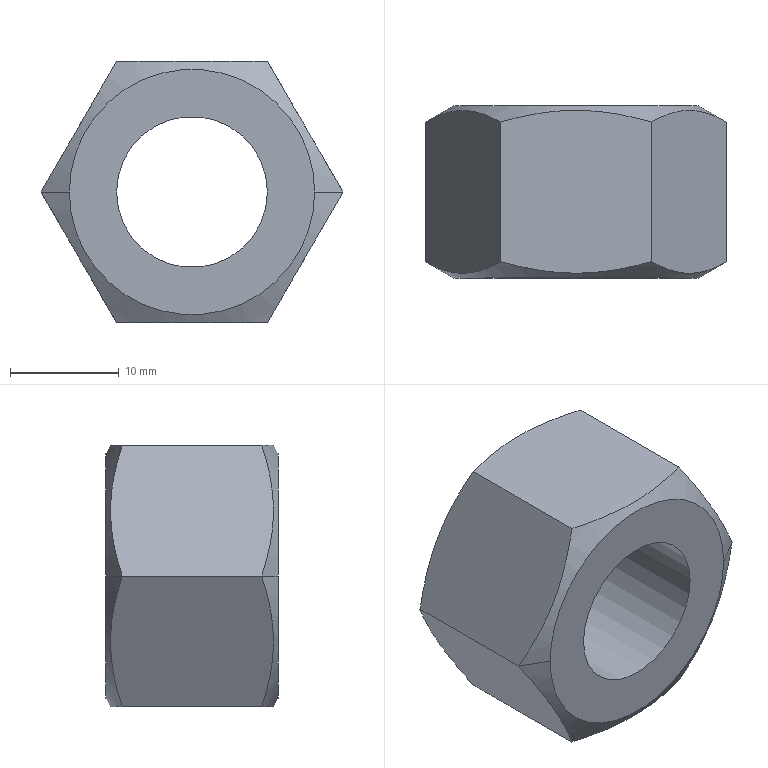Component | SolidWorks | m16-3 | 1 solid | 14 faces | box 27.71 x 15.8 x 24 mm | volume 5411 mm3 | plane 8 | cone 4 | cylinder 2 | commonest cylinder face diameters 13.84 x2
build123d program:
from build123d import *

# Parameters (mm, degrees)
BOSS_EXTRUDE1_DEPTH = 15.8
SKETCH3_R           = 6.92
CUT_EXTRUDE1_DEPTH  = 25.2


with BuildPart() as part:
    # Sketch1 → Boss-Extrude1 (new body)
    with BuildSketch(Plane.XY):
        Polygon((13.856, 0), (6.928, 12), (-6.928, 12), (-13.856, 0), (-6.928, -12), (6.928, -12), align=None)
    extrude(amount=BOSS_EXTRUDE1_DEPTH)

    # Sketch2 → Cut-Revolve1 (revolve, cut)
    with BuildSketch(Plane(origin=(0, 0, 0), x_dir=(1, 0, 0), z_dir=(0, 1, 0))):
        Polygon((13.856, -1.5), (6.928, 2.5), (16.856, 3.696), align=None)
        Polygon((13.856, -14.3), (6.928, -18.3), (16.856, -19.496), align=None)
    revolve(axis=Axis((0, 0, 0), (0, 0, 1)), mode=Mode.SUBTRACT)

    # Sketch3 → Cut-Extrude1 (cut, through all)
    with BuildSketch(Plane.XY):
        Circle(SKETCH3_R)
    extrude(amount=CUT_EXTRUDE1_DEPTH, mode=Mode.SUBTRACT)


solid = part.part

# Placed as in the assembly
solid = solid.moved(Location((726.83, 1299.391, 1682.217), (90, 0, 0)))
STEP:
#1=COLOUR_RGB('',0.7922,0.8196,0.9333);
#2=FILL_AREA_STYLE_COLOUR('',#1);
#3=FILL_AREA_STYLE('',(#2));
#4=SURFACE_STYLE_FILL_AREA(#3);
#5=SURFACE_SIDE_STYLE('',(#4));
#6=SURFACE_STYLE_USAGE(.BOTH.,#5);
#7=PRESENTATION_STYLE_ASSIGNMENT((#6));
#8=CARTESIAN_POINT('',(28.343,50.535,66.229));
#9=VERTEX_POINT('',#8);
#10=CARTESIAN_POINT('',(28.888,50.535,66.229));
#11=VERTEX_POINT('',#10);
#12=CARTESIAN_POINT('',(28.615,50.535,66.229));
#13=DIRECTION('',(0.,-1.,0.));
#14=DIRECTION('',(1.,0.,0.));
#15=AXIS2_PLACEMENT_3D('',#12,#13,#14);
#16=CIRCLE('',#15,0.2724);
#17=EDGE_CURVE('',#9,#11,#16,.T.);
#18=ORIENTED_EDGE('',*,*,#17,.T.);
#19=CARTESIAN_POINT('',(28.888,51.157,66.229));
#20=VERTEX_POINT('',#19);
#21=CARTESIAN_POINT('',(28.888,50.535,66.229));
#22=DIRECTION('',(0.,1.,0.));
#23=VECTOR('',#22,39.37);
#24=LINE('',#21,#23);
#25=EDGE_CURVE('',#11,#20,#24,.T.);
#26=ORIENTED_EDGE('',*,*,#25,.T.);
#27=CARTESIAN_POINT('',(28.343,51.157,66.229));
#28=VERTEX_POINT('',#27);
#29=CARTESIAN_POINT('',(28.615,51.157,66.229));
#30=DIRECTION('',(0.,-1.,0.));
#31=DIRECTION('',(1.,0.,0.));
#32=AXIS2_PLACEMENT_3D('',#29,#30,#31);
#33=CIRCLE('',#32,0.2724);
#34=EDGE_CURVE('',#28,#20,#33,.T.);
#35=ORIENTED_EDGE('',*,*,#34,.F.);
#36=CARTESIAN_POINT('',(28.343,50.535,66.229));
#37=DIRECTION('',(0.,1.,0.));
#38=VECTOR('',#37,39.37);
#39=LINE('',#36,#38);
#40=EDGE_CURVE('',#9,#28,#39,.T.);
#41=ORIENTED_EDGE('',*,*,#40,.F.);
#42=EDGE_LOOP('',(#18,#26,#35,#41));
#43=FACE_OUTER_BOUND('',#42,.T.);
#44=CARTESIAN_POINT('',(28.615,50.535,66.229));
#45=DIRECTION('',(0.,1.,0.));
#46=DIRECTION('',(-1.,0.,0.));
#47=AXIS2_PLACEMENT_3D('',#44,#45,#46);
#48=CYLINDRICAL_SURFACE('',#47,0.2724);
#49=ADVANCED_FACE('',(#43),#48,.F.);
#50=CARTESIAN_POINT('',(29.059,51.157,66.229));
#51=VERTEX_POINT('',#50);
#52=CARTESIAN_POINT('',(28.172,51.157,66.229));
#53=VERTEX_POINT('',#52);
#54=CARTESIAN_POINT('',(28.615,51.157,66.229));
#55=DIRECTION('',(0.,-1.,0.));
#56=DIRECTION('',(1.,0.,0.));
#57=AXIS2_PLACEMENT_3D('',#54,#55,#56);
#58=CIRCLE('',#57,0.4432);
#59=EDGE_CURVE('',#51,#53,#58,.T.);
#60=ORIENTED_EDGE('',*,*,#59,.T.);
#61=CARTESIAN_POINT('',(28.07,51.098,66.229));
#62=VERTEX_POINT('',#61);
#63=CARTESIAN_POINT('',(28.343,51.256,66.229));
#64=DIRECTION('',(-0.866,-0.5,0.));
#65=VECTOR('',#64,39.37);
#66=LINE('',#63,#65);
#67=EDGE_CURVE('',#53,#62,#66,.T.);
#68=ORIENTED_EDGE('',*,*,#67,.T.);
#69=CARTESIAN_POINT('',(28.343,51.098,66.701));
#70=VERTEX_POINT('',#69);
#71=CARTESIAN_POINT('',(28.07,51.098,66.229));
#72=CARTESIAN_POINT('',(28.092,51.111,66.268));
#73=CARTESIAN_POINT('',(28.115,51.122,66.306));
#74=CARTESIAN_POINT('',(28.16,51.136,66.385));
#75=CARTESIAN_POINT('',(28.183,51.14,66.425));
#76=CARTESIAN_POINT('',(28.218,51.14,66.485));
#77=CARTESIAN_POINT('',(28.229,51.139,66.505));
#78=CARTESIAN_POINT('',(28.252,51.135,66.545));
#79=CARTESIAN_POINT('',(28.264,51.133,66.565));
#80=CARTESIAN_POINT('',(28.298,51.122,66.624));
#81=CARTESIAN_POINT('',(28.32,51.111,66.663));
#82=CARTESIAN_POINT('',(28.343,51.098,66.701));
#83=B_SPLINE_CURVE_WITH_KNOTS('',3,(#71,#72,#73,#74,#75,#76,#77,#78,#79,#80,#81,#82),.UNSPECIFIED.,.F.,.F.,(4,2,2,2,2,4),(0.00000024,0.003499,0.006997,0.008747,0.0105,0.01399),.UNSPECIFIED.);
#84=EDGE_CURVE('',#62,#70,#83,.T.);
#85=ORIENTED_EDGE('',*,*,#84,.T.);
#86=CARTESIAN_POINT('',(28.888,51.098,66.701));
#87=VERTEX_POINT('',#86);
#88=CARTESIAN_POINT('',(28.343,51.098,66.701));
#89=CARTESIAN_POINT('',(28.387,51.111,66.701));
#90=CARTESIAN_POINT('',(28.432,51.121,66.701));
#91=CARTESIAN_POINT('',(28.523,51.136,66.701));
#92=CARTESIAN_POINT('',(28.569,51.14,66.701));
#93=CARTESIAN_POINT('',(28.662,51.14,66.701));
#94=CARTESIAN_POINT('',(28.708,51.136,66.701));
#95=CARTESIAN_POINT('',(28.799,51.121,66.701));
#96=CARTESIAN_POINT('',(28.844,51.111,66.701));
#97=CARTESIAN_POINT('',(28.888,51.098,66.701));
#98=B_SPLINE_CURVE_WITH_KNOTS('',3,(#88,#89,#90,#91,#92,#93,#94,#95,#96,#97),.UNSPECIFIED.,.F.,.F.,(4,2,2,2,4),(0.01514,0.01866,0.02219,0.02571,0.02923),.UNSPECIFIED.);
#99=EDGE_CURVE('',#70,#87,#98,.T.);
#100=ORIENTED_EDGE('',*,*,#99,.T.);
#101=CARTESIAN_POINT('',(29.161,51.098,66.229));
#102=VERTEX_POINT('',#101);
#103=CARTESIAN_POINT('',(28.888,51.098,66.701));
#104=CARTESIAN_POINT('',(28.91,51.111,66.663));
#105=CARTESIAN_POINT('',(28.933,51.122,66.624));
#106=CARTESIAN_POINT('',(28.978,51.136,66.546));
#107=CARTESIAN_POINT('',(29.001,51.14,66.506));
#108=CARTESIAN_POINT('',(29.036,51.14,66.446));
#109=CARTESIAN_POINT('',(29.047,51.139,66.425));
#110=CARTESIAN_POINT('',(29.071,51.135,66.386));
#111=CARTESIAN_POINT('',(29.082,51.133,66.366));
#112=CARTESIAN_POINT('',(29.116,51.122,66.307));
#113=CARTESIAN_POINT('',(29.139,51.111,66.268));
#114=CARTESIAN_POINT('',(29.161,51.098,66.229));
#115=B_SPLINE_CURVE_WITH_KNOTS('',3,(#103,#104,#105,#106,#107,#108,#109,#110,#111,#112,#113,#114),.UNSPECIFIED.,.F.,.F.,(4,2,2,2,2,4),(0.00000024,0.003499,0.006997,0.008747,0.0105,0.01399),.UNSPECIFIED.);
#116=EDGE_CURVE('',#87,#102,#115,.T.);
#117=ORIENTED_EDGE('',*,*,#116,.T.);
#118=CARTESIAN_POINT('',(28.888,51.256,66.229));
#119=DIRECTION('',(0.866,-0.5,0.));
#120=VECTOR('',#119,39.37);
#121=LINE('',#118,#120);
#122=EDGE_CURVE('',#51,#102,#121,.T.);
#123=ORIENTED_EDGE('',*,*,#122,.F.);
#124=EDGE_LOOP('',(#60,#68,#85,#100,#117,#123));
#125=FACE_OUTER_BOUND('',#124,.T.);
#126=CARTESIAN_POINT('',(28.615,51.256,66.229));
#127=DIRECTION('',(-0.,-1.,0.));
#128=DIRECTION('',(1.,0.,0.));
#129=AXIS2_PLACEMENT_3D('',#126,#127,#128);
#130=CONICAL_SURFACE('',#129,0.2728,1.047);
#131=ADVANCED_FACE('',(#125),#130,.T.);
#132=CARTESIAN_POINT('',(29.059,50.535,66.229));
#133=VERTEX_POINT('',#132);
#134=CARTESIAN_POINT('',(28.172,50.535,66.229));
#135=VERTEX_POINT('',#134);
#136=CARTESIAN_POINT('',(28.615,50.535,66.229));
#137=DIRECTION('',(0.,-1.,0.));
#138=DIRECTION('',(1.,0.,0.));
#139=AXIS2_PLACEMENT_3D('',#136,#137,#138);
#140=CIRCLE('',#139,0.4432);
#141=EDGE_CURVE('',#133,#135,#140,.T.);
#142=ORIENTED_EDGE('',*,*,#141,.F.);
#143=CARTESIAN_POINT('',(29.161,50.594,66.229));
#144=VERTEX_POINT('',#143);
#145=CARTESIAN_POINT('',(29.161,50.594,66.229));
#146=DIRECTION('',(0.866,0.5,0.));
#147=VECTOR('',#146,39.37);
#148=LINE('',#145,#147);
#149=EDGE_CURVE('',#133,#144,#148,.T.);
#150=ORIENTED_EDGE('',*,*,#149,.T.);
#151=CARTESIAN_POINT('',(28.888,50.594,66.701));
#152=VERTEX_POINT('',#151);
#153=CARTESIAN_POINT('',(29.161,50.594,66.229));
#154=CARTESIAN_POINT('',(29.139,50.581,66.268));
#155=CARTESIAN_POINT('',(29.116,50.571,66.306));
#156=CARTESIAN_POINT('',(29.071,50.556,66.385));
#157=CARTESIAN_POINT('',(29.048,50.552,66.425));
#158=CARTESIAN_POINT('',(29.013,50.552,66.485));
#159=CARTESIAN_POINT('',(29.002,50.553,66.505));
#160=CARTESIAN_POINT('',(28.978,50.557,66.545));
#161=CARTESIAN_POINT('',(28.967,50.56,66.565));
#162=CARTESIAN_POINT('',(28.933,50.571,66.624));
#163=CARTESIAN_POINT('',(28.91,50.581,66.663));
#164=CARTESIAN_POINT('',(28.888,50.594,66.701));
#165=B_SPLINE_CURVE_WITH_KNOTS('',3,(#153,#154,#155,#156,#157,#158,#159,#160,#161,#162,#163,#164),.UNSPECIFIED.,.F.,.F.,(4,2,2,2,2,4),(0.00000024,0.003499,0.006997,0.008747,0.0105,0.01399),.UNSPECIFIED.);
#166=EDGE_CURVE('',#144,#152,#165,.T.);
#167=ORIENTED_EDGE('',*,*,#166,.T.);
#168=CARTESIAN_POINT('',(28.343,50.594,66.701));
#169=VERTEX_POINT('',#168);
#170=CARTESIAN_POINT('',(28.888,50.594,66.701));
#171=CARTESIAN_POINT('',(28.844,50.581,66.701));
#172=CARTESIAN_POINT('',(28.799,50.571,66.701));
#173=CARTESIAN_POINT('',(28.708,50.556,66.701));
#174=CARTESIAN_POINT('',(28.662,50.552,66.701));
#175=CARTESIAN_POINT('',(28.569,50.552,66.701));
#176=CARTESIAN_POINT('',(28.523,50.556,66.701));
#177=CARTESIAN_POINT('',(28.432,50.571,66.701));
#178=CARTESIAN_POINT('',(28.387,50.581,66.701));
#179=CARTESIAN_POINT('',(28.343,50.594,66.701));
#180=B_SPLINE_CURVE_WITH_KNOTS('',3,(#170,#171,#172,#173,#174,#175,#176,#177,#178,#179),.UNSPECIFIED.,.F.,.F.,(4,2,2,2,4),(0.01514,0.01866,0.02219,0.02571,0.02923),.UNSPECIFIED.);
#181=EDGE_CURVE('',#152,#169,#180,.T.);
#182=ORIENTED_EDGE('',*,*,#181,.T.);
#183=CARTESIAN_POINT('',(28.07,50.594,66.229));
#184=VERTEX_POINT('',#183);
#185=CARTESIAN_POINT('',(28.343,50.594,66.701));
#186=CARTESIAN_POINT('',(28.32,50.581,66.663));
#187=CARTESIAN_POINT('',(28.298,50.571,66.624));
#188=CARTESIAN_POINT('',(28.253,50.556,66.546));
#189=CARTESIAN_POINT('',(28.23,50.552,66.506));
#190=CARTESIAN_POINT('',(28.195,50.552,66.446));
#191=CARTESIAN_POINT('',(28.183,50.553,66.425));
#192=CARTESIAN_POINT('',(28.16,50.557,66.386));
#193=CARTESIAN_POINT('',(28.149,50.56,66.366));
#194=CARTESIAN_POINT('',(28.115,50.571,66.307));
#195=CARTESIAN_POINT('',(28.092,50.581,66.268));
#196=CARTESIAN_POINT('',(28.07,50.594,66.229));
#197=B_SPLINE_CURVE_WITH_KNOTS('',3,(#185,#186,#187,#188,#189,#190,#191,#192,#193,#194,#195,#196),.UNSPECIFIED.,.F.,.F.,(4,2,2,2,2,4),(0.00000024,0.003499,0.006997,0.008747,0.0105,0.01399),.UNSPECIFIED.);
#198=EDGE_CURVE('',#169,#184,#197,.T.);
#199=ORIENTED_EDGE('',*,*,#198,.T.);
#200=CARTESIAN_POINT('',(28.07,50.594,66.229));
#201=DIRECTION('',(-0.866,0.5,0.));
#202=VECTOR('',#201,39.37);
#203=LINE('',#200,#202);
#204=EDGE_CURVE('',#135,#184,#203,.T.);
#205=ORIENTED_EDGE('',*,*,#204,.F.);
#206=EDGE_LOOP('',(#142,#150,#167,#182,#199,#205));
#207=FACE_OUTER_BOUND('',#206,.T.);
#208=CARTESIAN_POINT('',(28.615,50.594,66.229));
#209=DIRECTION('',(0.,1.,0.));
#210=DIRECTION('',(-1.,0.,0.));
#211=AXIS2_PLACEMENT_3D('',#208,#209,#210);
#212=CONICAL_SURFACE('',#211,0.5455,1.047);
#213=ADVANCED_FACE('',(#207),#212,.T.);
#214=ORIENTED_EDGE('',*,*,#17,.F.);
#215=CARTESIAN_POINT('',(28.615,50.535,66.229));
#216=DIRECTION('',(0.,-1.,0.));
#217=DIRECTION('',(1.,0.,0.));
#218=AXIS2_PLACEMENT_3D('',#215,#216,#217);
#219=CIRCLE('',#218,0.2724);
#220=EDGE_CURVE('',#11,#9,#219,.T.);
#221=ORIENTED_EDGE('',*,*,#220,.F.);
#222=EDGE_LOOP('',(#214,#221));
#223=FACE_BOUND('',#222,.T.);
#224=CARTESIAN_POINT('',(28.615,50.535,66.229));
#225=DIRECTION('',(0.,-1.,0.));
#226=DIRECTION('',(1.,0.,0.));
#227=AXIS2_PLACEMENT_3D('',#224,#225,#226);
#228=CIRCLE('',#227,0.4432);
#229=EDGE_CURVE('',#135,#133,#228,.T.);
#230=ORIENTED_EDGE('',*,*,#229,.T.);
#231=ORIENTED_EDGE('',*,*,#141,.T.);
#232=EDGE_LOOP('',(#230,#231));
#233=FACE_OUTER_BOUND('',#232,.T.);
#234=CARTESIAN_POINT('',(28.615,50.535,66.229));
#235=DIRECTION('',(0.,-1.,0.));
#236=DIRECTION('',(1.,0.,0.));
#237=AXIS2_PLACEMENT_3D('',#234,#235,#236);
#238=PLANE('',#237);
#239=ADVANCED_FACE('',(#223,#233),#238,.T.);
#240=ORIENTED_EDGE('',*,*,#149,.F.);
#241=ORIENTED_EDGE('',*,*,#229,.F.);
#242=ORIENTED_EDGE('',*,*,#204,.T.);
#243=CARTESIAN_POINT('',(28.343,50.594,65.757));
#244=VERTEX_POINT('',#243);
#245=CARTESIAN_POINT('',(28.07,50.594,66.229));
#246=CARTESIAN_POINT('',(28.092,50.581,66.19));
#247=CARTESIAN_POINT('',(28.115,50.571,66.152));
#248=CARTESIAN_POINT('',(28.16,50.556,66.073));
#249=CARTESIAN_POINT('',(28.183,50.552,66.033));
#250=CARTESIAN_POINT('',(28.218,50.552,65.973));
#251=CARTESIAN_POINT('',(28.229,50.553,65.953));
#252=CARTESIAN_POINT('',(28.252,50.557,65.913));
#253=CARTESIAN_POINT('',(28.264,50.56,65.893));
#254=CARTESIAN_POINT('',(28.298,50.571,65.834));
#255=CARTESIAN_POINT('',(28.32,50.581,65.795));
#256=CARTESIAN_POINT('',(28.343,50.594,65.757));
#257=B_SPLINE_CURVE_WITH_KNOTS('',3,(#245,#246,#247,#248,#249,#250,#251,#252,#253,#254,#255,#256),.UNSPECIFIED.,.F.,.F.,(4,2,2,2,2,4),(0.00000024,0.003499,0.006997,0.008747,0.0105,0.01399),.UNSPECIFIED.);
#258=EDGE_CURVE('',#184,#244,#257,.T.);
#259=ORIENTED_EDGE('',*,*,#258,.T.);
#260=CARTESIAN_POINT('',(28.888,50.594,65.757));
#261=VERTEX_POINT('',#260);
#262=CARTESIAN_POINT('',(28.343,50.594,65.757));
#263=CARTESIAN_POINT('',(28.387,50.581,65.757));
#264=CARTESIAN_POINT('',(28.432,50.571,65.757));
#265=CARTESIAN_POINT('',(28.523,50.556,65.757));
#266=CARTESIAN_POINT('',(28.569,50.552,65.757));
#267=CARTESIAN_POINT('',(28.662,50.552,65.757));
#268=CARTESIAN_POINT('',(28.708,50.556,65.757));
#269=CARTESIAN_POINT('',(28.799,50.571,65.757));
#270=CARTESIAN_POINT('',(28.844,50.581,65.757));
#271=CARTESIAN_POINT('',(28.888,50.594,65.757));
#272=B_SPLINE_CURVE_WITH_KNOTS('',3,(#262,#263,#264,#265,#266,#267,#268,#269,#270,#271),.UNSPECIFIED.,.F.,.F.,(4,2,2,2,4),(0.01514,0.01866,0.02219,0.02571,0.02923),.UNSPECIFIED.);
#273=EDGE_CURVE('',#244,#261,#272,.T.);
#274=ORIENTED_EDGE('',*,*,#273,.T.);
#275=CARTESIAN_POINT('',(28.888,50.594,65.757));
#276=CARTESIAN_POINT('',(28.91,50.581,65.795));
#277=CARTESIAN_POINT('',(28.933,50.571,65.834));
#278=CARTESIAN_POINT('',(28.978,50.556,65.912));
#279=CARTESIAN_POINT('',(29.001,50.552,65.952));
#280=CARTESIAN_POINT('',(29.036,50.552,66.012));
#281=CARTESIAN_POINT('',(29.047,50.553,66.033));
#282=CARTESIAN_POINT('',(29.071,50.557,66.073));
#283=CARTESIAN_POINT('',(29.082,50.56,66.092));
#284=CARTESIAN_POINT('',(29.116,50.571,66.151));
#285=CARTESIAN_POINT('',(29.139,50.581,66.19));
#286=CARTESIAN_POINT('',(29.161,50.594,66.229));
#287=B_SPLINE_CURVE_WITH_KNOTS('',3,(#275,#276,#277,#278,#279,#280,#281,#282,#283,#284,#285,#286),.UNSPECIFIED.,.F.,.F.,(4,2,2,2,2,4),(0.00000024,0.003499,0.006997,0.008747,0.0105,0.01399),.UNSPECIFIED.);
#288=EDGE_CURVE('',#261,#144,#287,.T.);
#289=ORIENTED_EDGE('',*,*,#288,.T.);
#290=EDGE_LOOP('',(#240,#241,#242,#259,#274,#289));
#291=FACE_OUTER_BOUND('',#290,.T.);
#292=CARTESIAN_POINT('',(28.615,50.594,66.229));
#293=DIRECTION('',(0.,1.,0.));
#294=DIRECTION('',(-1.,0.,0.));
#295=AXIS2_PLACEMENT_3D('',#292,#293,#294);
#296=CONICAL_SURFACE('',#295,0.5455,1.047);
#297=ADVANCED_FACE('',(#291),#296,.T.);
#298=CARTESIAN_POINT('',(28.888,51.098,65.757));
#299=VERTEX_POINT('',#298);
#300=CARTESIAN_POINT('',(29.161,51.098,66.229));
#301=CARTESIAN_POINT('',(29.139,51.111,66.19));
#302=CARTESIAN_POINT('',(29.116,51.122,66.152));
#303=CARTESIAN_POINT('',(29.071,51.136,66.073));
#304=CARTESIAN_POINT('',(29.048,51.14,66.033));
#305=CARTESIAN_POINT('',(29.013,51.14,65.973));
#306=CARTESIAN_POINT('',(29.002,51.139,65.953));
#307=CARTESIAN_POINT('',(28.978,51.135,65.913));
#308=CARTESIAN_POINT('',(28.967,51.133,65.893));
#309=CARTESIAN_POINT('',(28.933,51.122,65.834));
#310=CARTESIAN_POINT('',(28.91,51.111,65.795));
#311=CARTESIAN_POINT('',(28.888,51.098,65.757));
#312=B_SPLINE_CURVE_WITH_KNOTS('',3,(#300,#301,#302,#303,#304,#305,#306,#307,#308,#309,#310,#311),.UNSPECIFIED.,.F.,.F.,(4,2,2,2,2,4),(0.00000024,0.003499,0.006997,0.008747,0.0105,0.01399),.UNSPECIFIED.);
#313=EDGE_CURVE('',#102,#299,#312,.T.);
#314=ORIENTED_EDGE('',*,*,#313,.F.);
#315=CARTESIAN_POINT('',(29.161,50.535,66.229));
#316=DIRECTION('',(0.,1.,0.));
#317=VECTOR('',#316,39.37);
#318=LINE('',#315,#317);
#319=EDGE_CURVE('',#144,#102,#318,.T.);
#320=ORIENTED_EDGE('',*,*,#319,.F.);
#321=ORIENTED_EDGE('',*,*,#288,.F.);
#322=CARTESIAN_POINT('',(28.888,50.535,65.757));
#323=DIRECTION('',(0.,1.,0.));
#324=VECTOR('',#323,39.37);
#325=LINE('',#322,#324);
#326=EDGE_CURVE('',#261,#299,#325,.T.);
#327=ORIENTED_EDGE('',*,*,#326,.T.);
#328=EDGE_LOOP('',(#314,#320,#321,#327));
#329=FACE_OUTER_BOUND('',#328,.T.);
#330=CARTESIAN_POINT('',(28.888,50.535,65.757));
#331=DIRECTION('',(-0.866,0.,0.5));
#332=DIRECTION('',(-0.5,0.,-0.866));
#333=AXIS2_PLACEMENT_3D('',#330,#331,#332);
#334=PLANE('',#333);
#335=ADVANCED_FACE('',(#329),#334,.F.);
#336=ORIENTED_EDGE('',*,*,#116,.F.);
#337=CARTESIAN_POINT('',(28.888,50.535,66.701));
#338=DIRECTION('',(0.,1.,0.));
#339=VECTOR('',#338,39.37);
#340=LINE('',#337,#339);
#341=EDGE_CURVE('',#152,#87,#340,.T.);
#342=ORIENTED_EDGE('',*,*,#341,.F.);
#343=ORIENTED_EDGE('',*,*,#166,.F.);
#344=ORIENTED_EDGE('',*,*,#319,.T.);
#345=EDGE_LOOP('',(#336,#342,#343,#344));
#346=FACE_OUTER_BOUND('',#345,.T.);
#347=CARTESIAN_POINT('',(29.161,50.535,66.229));
#348=DIRECTION('',(-0.866,0.,-0.5));
#349=DIRECTION('',(0.5,0.,-0.866));
#350=AXIS2_PLACEMENT_3D('',#347,#348,#349);
#351=PLANE('',#350);
#352=ADVANCED_FACE('',(#346),#351,.F.);
#353=ORIENTED_EDGE('',*,*,#99,.F.);
#354=CARTESIAN_POINT('',(28.343,50.535,66.701));
#355=DIRECTION('',(0.,1.,0.));
#356=VECTOR('',#355,39.37);
#357=LINE('',#354,#356);
#358=EDGE_CURVE('',#169,#70,#357,.T.);
#359=ORIENTED_EDGE('',*,*,#358,.F.);
#360=ORIENTED_EDGE('',*,*,#181,.F.);
#361=ORIENTED_EDGE('',*,*,#341,.T.);
#362=EDGE_LOOP('',(#353,#359,#360,#361));
#363=FACE_OUTER_BOUND('',#362,.T.);
#364=CARTESIAN_POINT('',(28.888,50.535,66.701));
#365=DIRECTION('',(0.,0.,-1.));
#366=DIRECTION('',(1.,0.,0.));
#367=AXIS2_PLACEMENT_3D('',#364,#365,#366);
#368=PLANE('',#367);
#369=ADVANCED_FACE('',(#363),#368,.F.);
#370=ORIENTED_EDGE('',*,*,#84,.F.);
#371=CARTESIAN_POINT('',(28.07,50.535,66.229));
#372=DIRECTION('',(0.,1.,0.));
#373=VECTOR('',#372,39.37);
#374=LINE('',#371,#373);
#375=EDGE_CURVE('',#184,#62,#374,.T.);
#376=ORIENTED_EDGE('',*,*,#375,.F.);
#377=ORIENTED_EDGE('',*,*,#198,.F.);
#378=ORIENTED_EDGE('',*,*,#358,.T.);
#379=EDGE_LOOP('',(#370,#376,#377,#378));
#380=FACE_OUTER_BOUND('',#379,.T.);
#381=CARTESIAN_POINT('',(28.343,50.535,66.701));
#382=DIRECTION('',(0.866,0.,-0.5));
#383=DIRECTION('',(0.5,0.,0.866));
#384=AXIS2_PLACEMENT_3D('',#381,#382,#383);
#385=PLANE('',#384);
#386=ADVANCED_FACE('',(#380),#385,.F.);
#387=CARTESIAN_POINT('',(28.343,51.098,65.757));
#388=VERTEX_POINT('',#387);
#389=CARTESIAN_POINT('',(28.343,51.098,65.757));
#390=CARTESIAN_POINT('',(28.32,51.111,65.795));
#391=CARTESIAN_POINT('',(28.298,51.122,65.834));
#392=CARTESIAN_POINT('',(28.253,51.136,65.912));
#393=CARTESIAN_POINT('',(28.23,51.14,65.952));
#394=CARTESIAN_POINT('',(28.195,51.14,66.012));
#395=CARTESIAN_POINT('',(28.183,51.139,66.033));
#396=CARTESIAN_POINT('',(28.16,51.135,66.073));
#397=CARTESIAN_POINT('',(28.149,51.133,66.092));
#398=CARTESIAN_POINT('',(28.115,51.122,66.151));
#399=CARTESIAN_POINT('',(28.092,51.111,66.19));
#400=CARTESIAN_POINT('',(28.07,51.098,66.229));
#401=B_SPLINE_CURVE_WITH_KNOTS('',3,(#389,#390,#391,#392,#393,#394,#395,#396,#397,#398,#399,#400),.UNSPECIFIED.,.F.,.F.,(4,2,2,2,2,4),(0.00000024,0.003499,0.006997,0.008747,0.0105,0.01399),.UNSPECIFIED.);
#402=EDGE_CURVE('',#388,#62,#401,.T.);
#403=ORIENTED_EDGE('',*,*,#402,.F.);
#404=CARTESIAN_POINT('',(28.343,50.535,65.757));
#405=DIRECTION('',(0.,1.,0.));
#406=VECTOR('',#405,39.37);
#407=LINE('',#404,#406);
#408=EDGE_CURVE('',#244,#388,#407,.T.);
#409=ORIENTED_EDGE('',*,*,#408,.F.);
#410=ORIENTED_EDGE('',*,*,#258,.F.);
#411=ORIENTED_EDGE('',*,*,#375,.T.);
#412=EDGE_LOOP('',(#403,#409,#410,#411));
#413=FACE_OUTER_BOUND('',#412,.T.);
#414=CARTESIAN_POINT('',(28.07,50.535,66.229));
#415=DIRECTION('',(0.866,0.,0.5));
#416=DIRECTION('',(-0.5,0.,0.866));
#417=AXIS2_PLACEMENT_3D('',#414,#415,#416);
#418=PLANE('',#417);
#419=ADVANCED_FACE('',(#413),#418,.F.);
#420=CARTESIAN_POINT('',(28.888,51.098,65.757));
#421=CARTESIAN_POINT('',(28.844,51.111,65.757));
#422=CARTESIAN_POINT('',(28.799,51.121,65.757));
#423=CARTESIAN_POINT('',(28.708,51.136,65.757));
#424=CARTESIAN_POINT('',(28.662,51.14,65.757));
#425=CARTESIAN_POINT('',(28.569,51.14,65.757));
#426=CARTESIAN_POINT('',(28.523,51.136,65.757));
#427=CARTESIAN_POINT('',(28.432,51.121,65.757));
#428=CARTESIAN_POINT('',(28.387,51.111,65.757));
#429=CARTESIAN_POINT('',(28.343,51.098,65.757));
#430=B_SPLINE_CURVE_WITH_KNOTS('',3,(#420,#421,#422,#423,#424,#425,#426,#427,#428,#429),.UNSPECIFIED.,.F.,.F.,(4,2,2,2,4),(0.01514,0.01866,0.02219,0.02571,0.02923),.UNSPECIFIED.);
#431=EDGE_CURVE('',#299,#388,#430,.T.);
#432=ORIENTED_EDGE('',*,*,#431,.F.);
#433=ORIENTED_EDGE('',*,*,#326,.F.);
#434=ORIENTED_EDGE('',*,*,#273,.F.);
#435=ORIENTED_EDGE('',*,*,#408,.T.);
#436=EDGE_LOOP('',(#432,#433,#434,#435));
#437=FACE_OUTER_BOUND('',#436,.T.);
#438=CARTESIAN_POINT('',(28.343,50.535,65.757));
#439=DIRECTION('',(-0.,0.,1.));
#440=DIRECTION('',(-1.,0.,-0.));
#441=AXIS2_PLACEMENT_3D('',#438,#439,#440);
#442=PLANE('',#441);
#443=ADVANCED_FACE('',(#437),#442,.F.);
#444=ORIENTED_EDGE('',*,*,#67,.F.);
#445=CARTESIAN_POINT('',(28.615,51.157,66.229));
#446=DIRECTION('',(0.,-1.,0.));
#447=DIRECTION('',(1.,0.,0.));
#448=AXIS2_PLACEMENT_3D('',#445,#446,#447);
#449=CIRCLE('',#448,0.4432);
#450=EDGE_CURVE('',#53,#51,#449,.T.);
#451=ORIENTED_EDGE('',*,*,#450,.T.);
#452=ORIENTED_EDGE('',*,*,#122,.T.);
#453=ORIENTED_EDGE('',*,*,#313,.T.);
#454=ORIENTED_EDGE('',*,*,#431,.T.);
#455=ORIENTED_EDGE('',*,*,#402,.T.);
#456=EDGE_LOOP('',(#444,#451,#452,#453,#454,#455));
#457=FACE_OUTER_BOUND('',#456,.T.);
#458=CARTESIAN_POINT('',(28.615,51.256,66.229));
#459=DIRECTION('',(-0.,-1.,0.));
#460=DIRECTION('',(1.,0.,0.));
#461=AXIS2_PLACEMENT_3D('',#458,#459,#460);
#462=CONICAL_SURFACE('',#461,0.2728,1.047);
#463=ADVANCED_FACE('',(#457),#462,.T.);
#464=ORIENTED_EDGE('',*,*,#34,.T.);
#465=CARTESIAN_POINT('',(28.615,51.157,66.229));
#466=DIRECTION('',(0.,-1.,0.));
#467=DIRECTION('',(1.,0.,0.));
#468=AXIS2_PLACEMENT_3D('',#465,#466,#467);
#469=CIRCLE('',#468,0.2724);
#470=EDGE_CURVE('',#20,#28,#469,.T.);
#471=ORIENTED_EDGE('',*,*,#470,.T.);
#472=EDGE_LOOP('',(#464,#471));
#473=FACE_BOUND('',#472,.T.);
#474=ORIENTED_EDGE('',*,*,#59,.F.);
#475=ORIENTED_EDGE('',*,*,#450,.F.);
#476=EDGE_LOOP('',(#474,#475));
#477=FACE_OUTER_BOUND('',#476,.T.);
#478=CARTESIAN_POINT('',(28.615,51.157,66.229));
#479=DIRECTION('',(0.,-1.,0.));
#480=DIRECTION('',(1.,0.,0.));
#481=AXIS2_PLACEMENT_3D('',#478,#479,#480);
#482=PLANE('',#481);
#483=ADVANCED_FACE('',(#473,#477),#482,.F.);
#484=ORIENTED_EDGE('',*,*,#25,.F.);
#485=ORIENTED_EDGE('',*,*,#220,.T.);
#486=ORIENTED_EDGE('',*,*,#40,.T.);
#487=ORIENTED_EDGE('',*,*,#470,.F.);
#488=EDGE_LOOP('',(#484,#485,#486,#487));
#489=FACE_OUTER_BOUND('',#488,.T.);
#490=CARTESIAN_POINT('',(28.615,50.535,66.229));
#491=DIRECTION('',(0.,1.,0.));
#492=DIRECTION('',(-1.,0.,0.));
#493=AXIS2_PLACEMENT_3D('',#490,#491,#492);
#494=CYLINDRICAL_SURFACE('',#493,0.2724);
#495=ADVANCED_FACE('',(#489),#494,.F.);
#496=CLOSED_SHELL('',(#49,#131,#213,#239,#297,#335,#352,#369,#386,#419,#443,#463,#483,#495));
#497=MANIFOLD_SOLID_BREP('',#496);
#498=STYLED_ITEM('',(#7),#497);
#499=(LENGTH_UNIT()NAMED_UNIT(*)SI_UNIT($,.METRE.));
#500=LENGTH_MEASURE_WITH_UNIT(LENGTH_MEASURE(0.0254),#499);
#501=DIMENSIONAL_EXPONENTS(1.,0.,0.,0.,0.,0.,0.);
#502=(CONVERSION_BASED_UNIT('',#500)LENGTH_UNIT()NAMED_UNIT(#501));
#503=UNCERTAINTY_MEASURE_WITH_UNIT(LENGTH_MEASURE(0.00001),#502,'','');
#504=(NAMED_UNIT(*)PLANE_ANGLE_UNIT()SI_UNIT($,.RADIAN.));
#505=(NAMED_UNIT(*)SI_UNIT($,.STERADIAN.)SOLID_ANGLE_UNIT());
#506=(GEOMETRIC_REPRESENTATION_CONTEXT(3)GLOBAL_UNCERTAINTY_ASSIGNED_CONTEXT((#503))GLOBAL_UNIT_ASSIGNED_CONTEXT((#502,#504,#505))REPRESENTATION_CONTEXT('',''));
#507=MECHANICAL_DESIGN_GEOMETRIC_PRESENTATION_REPRESENTATION('',(#498),#506);
#508=PRESENTATION_LAYER_ASSIGNMENT('','',(#498));
#509=CARTESIAN_POINT('',(0.,0.,0.));
#510=DIRECTION('',(0.,0.,1.));
#511=DIRECTION('',(1.,0.,0.));
#512=AXIS2_PLACEMENT_3D('',#509,#510,#511);
#513=(LENGTH_UNIT()NAMED_UNIT(*)SI_UNIT($,.METRE.));
#514=LENGTH_MEASURE_WITH_UNIT(LENGTH_MEASURE(0.0254),#513);
#515=DIMENSIONAL_EXPONENTS(1.,0.,0.,0.,0.,0.,0.);
#516=(CONVERSION_BASED_UNIT('',#514)LENGTH_UNIT()NAMED_UNIT(#515));
#517=UNCERTAINTY_MEASURE_WITH_UNIT(LENGTH_MEASURE(0.00001),#516,'','');
#518=(NAMED_UNIT(*)PLANE_ANGLE_UNIT()SI_UNIT($,.RADIAN.));
#519=(NAMED_UNIT(*)SI_UNIT($,.STERADIAN.)SOLID_ANGLE_UNIT());
#520=(GEOMETRIC_REPRESENTATION_CONTEXT(3)GLOBAL_UNCERTAINTY_ASSIGNED_CONTEXT((#517))GLOBAL_UNIT_ASSIGNED_CONTEXT((#516,#518,#519))REPRESENTATION_CONTEXT('',''));
#521=ADVANCED_BREP_SHAPE_REPRESENTATION('',(#497,#512),#520);